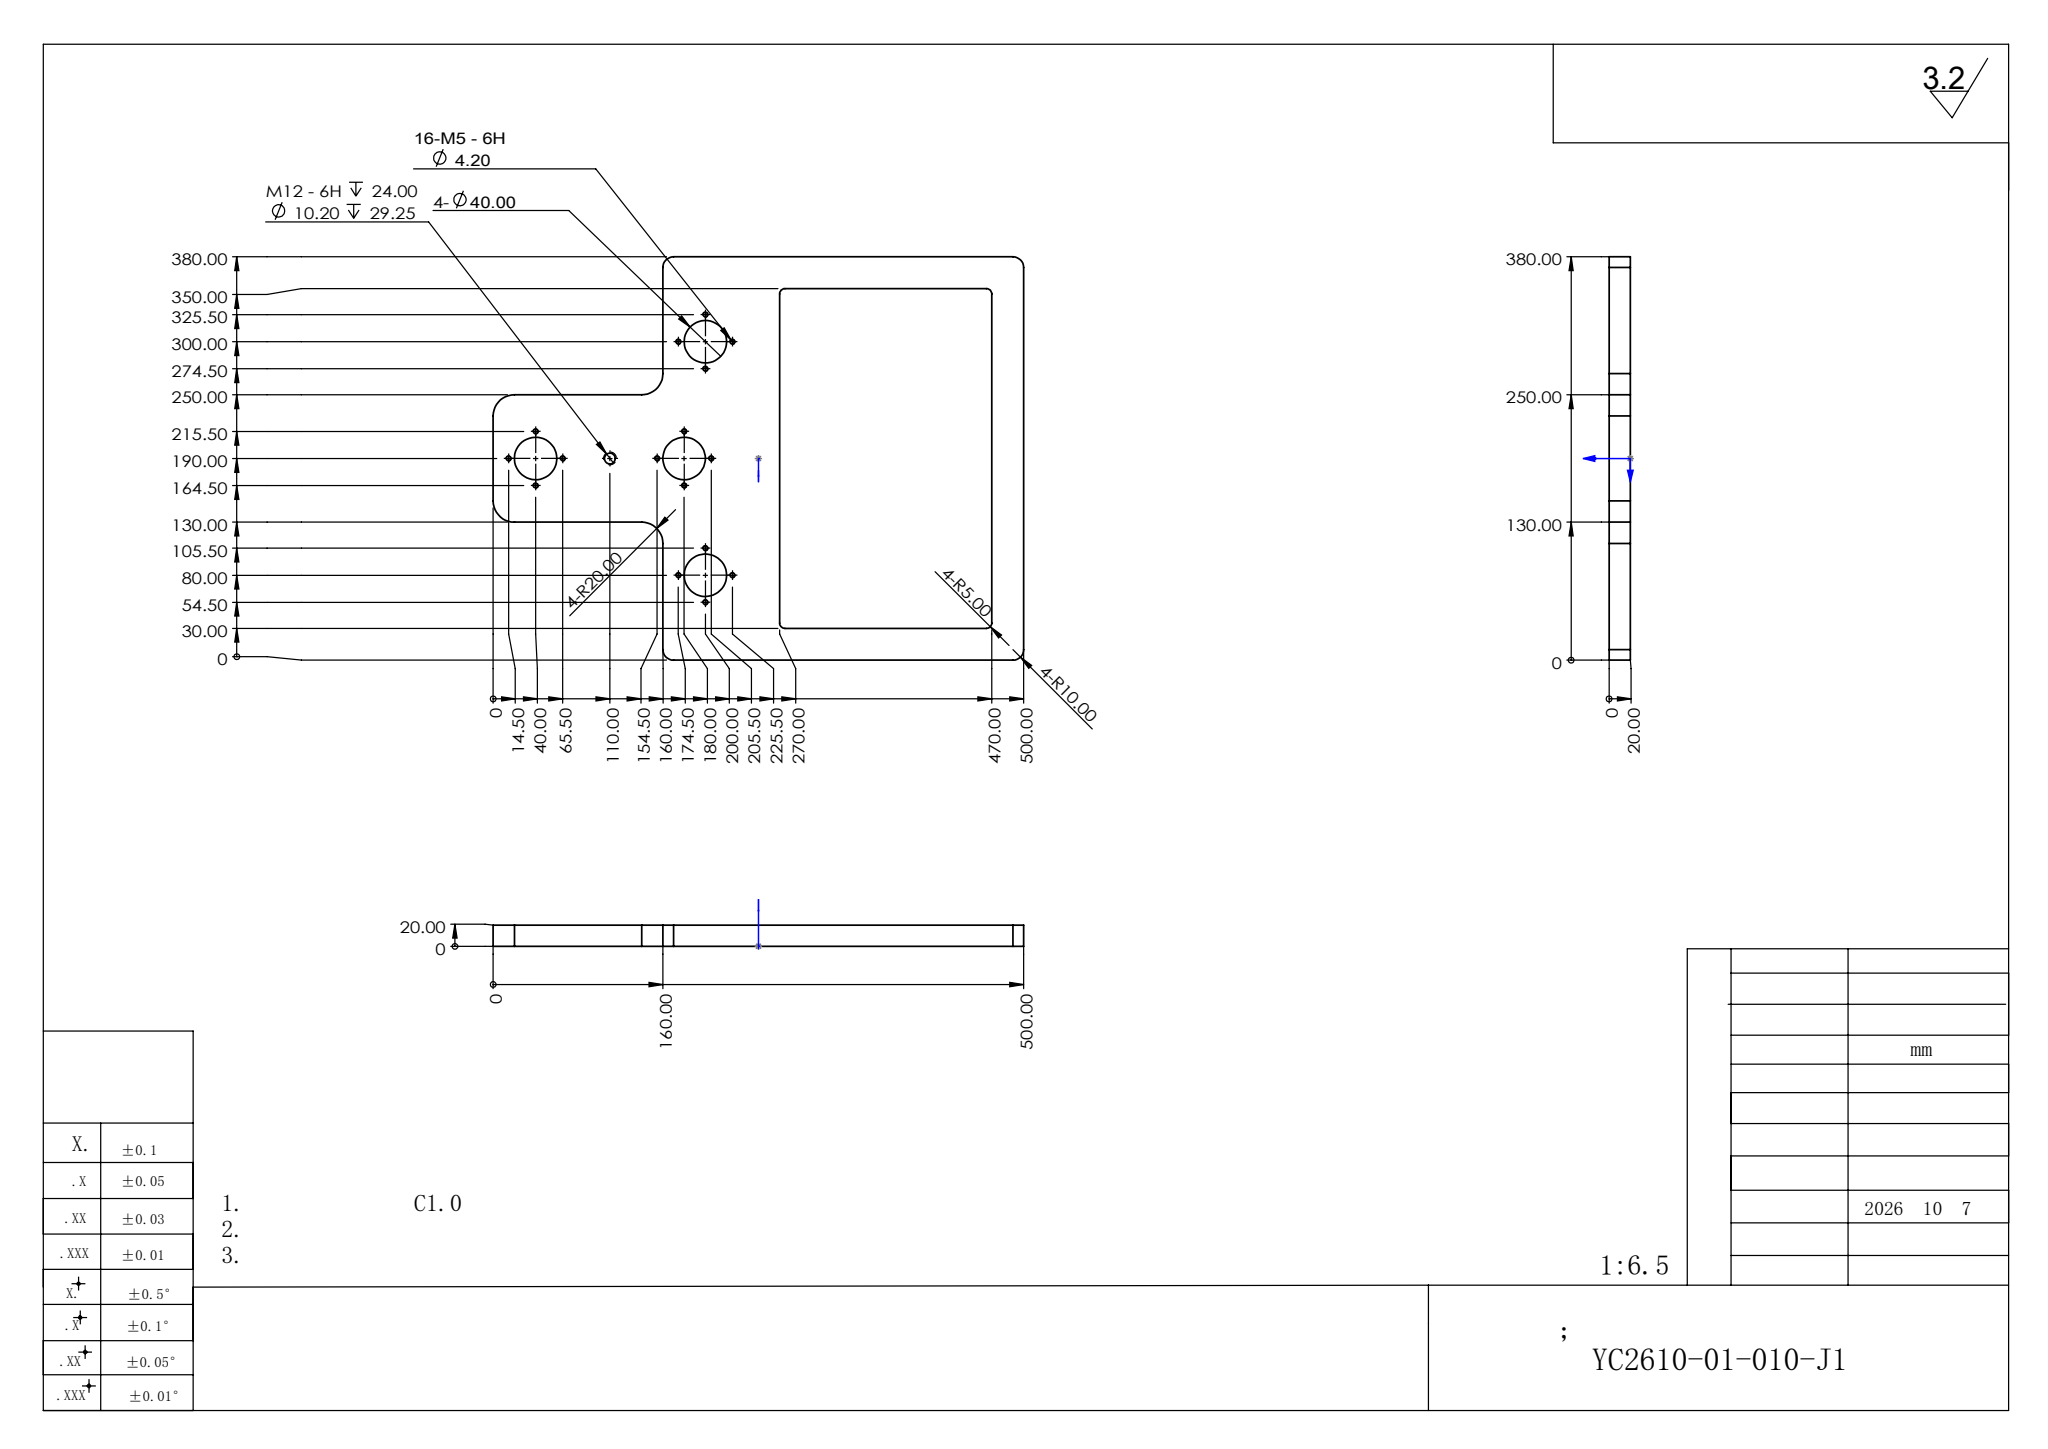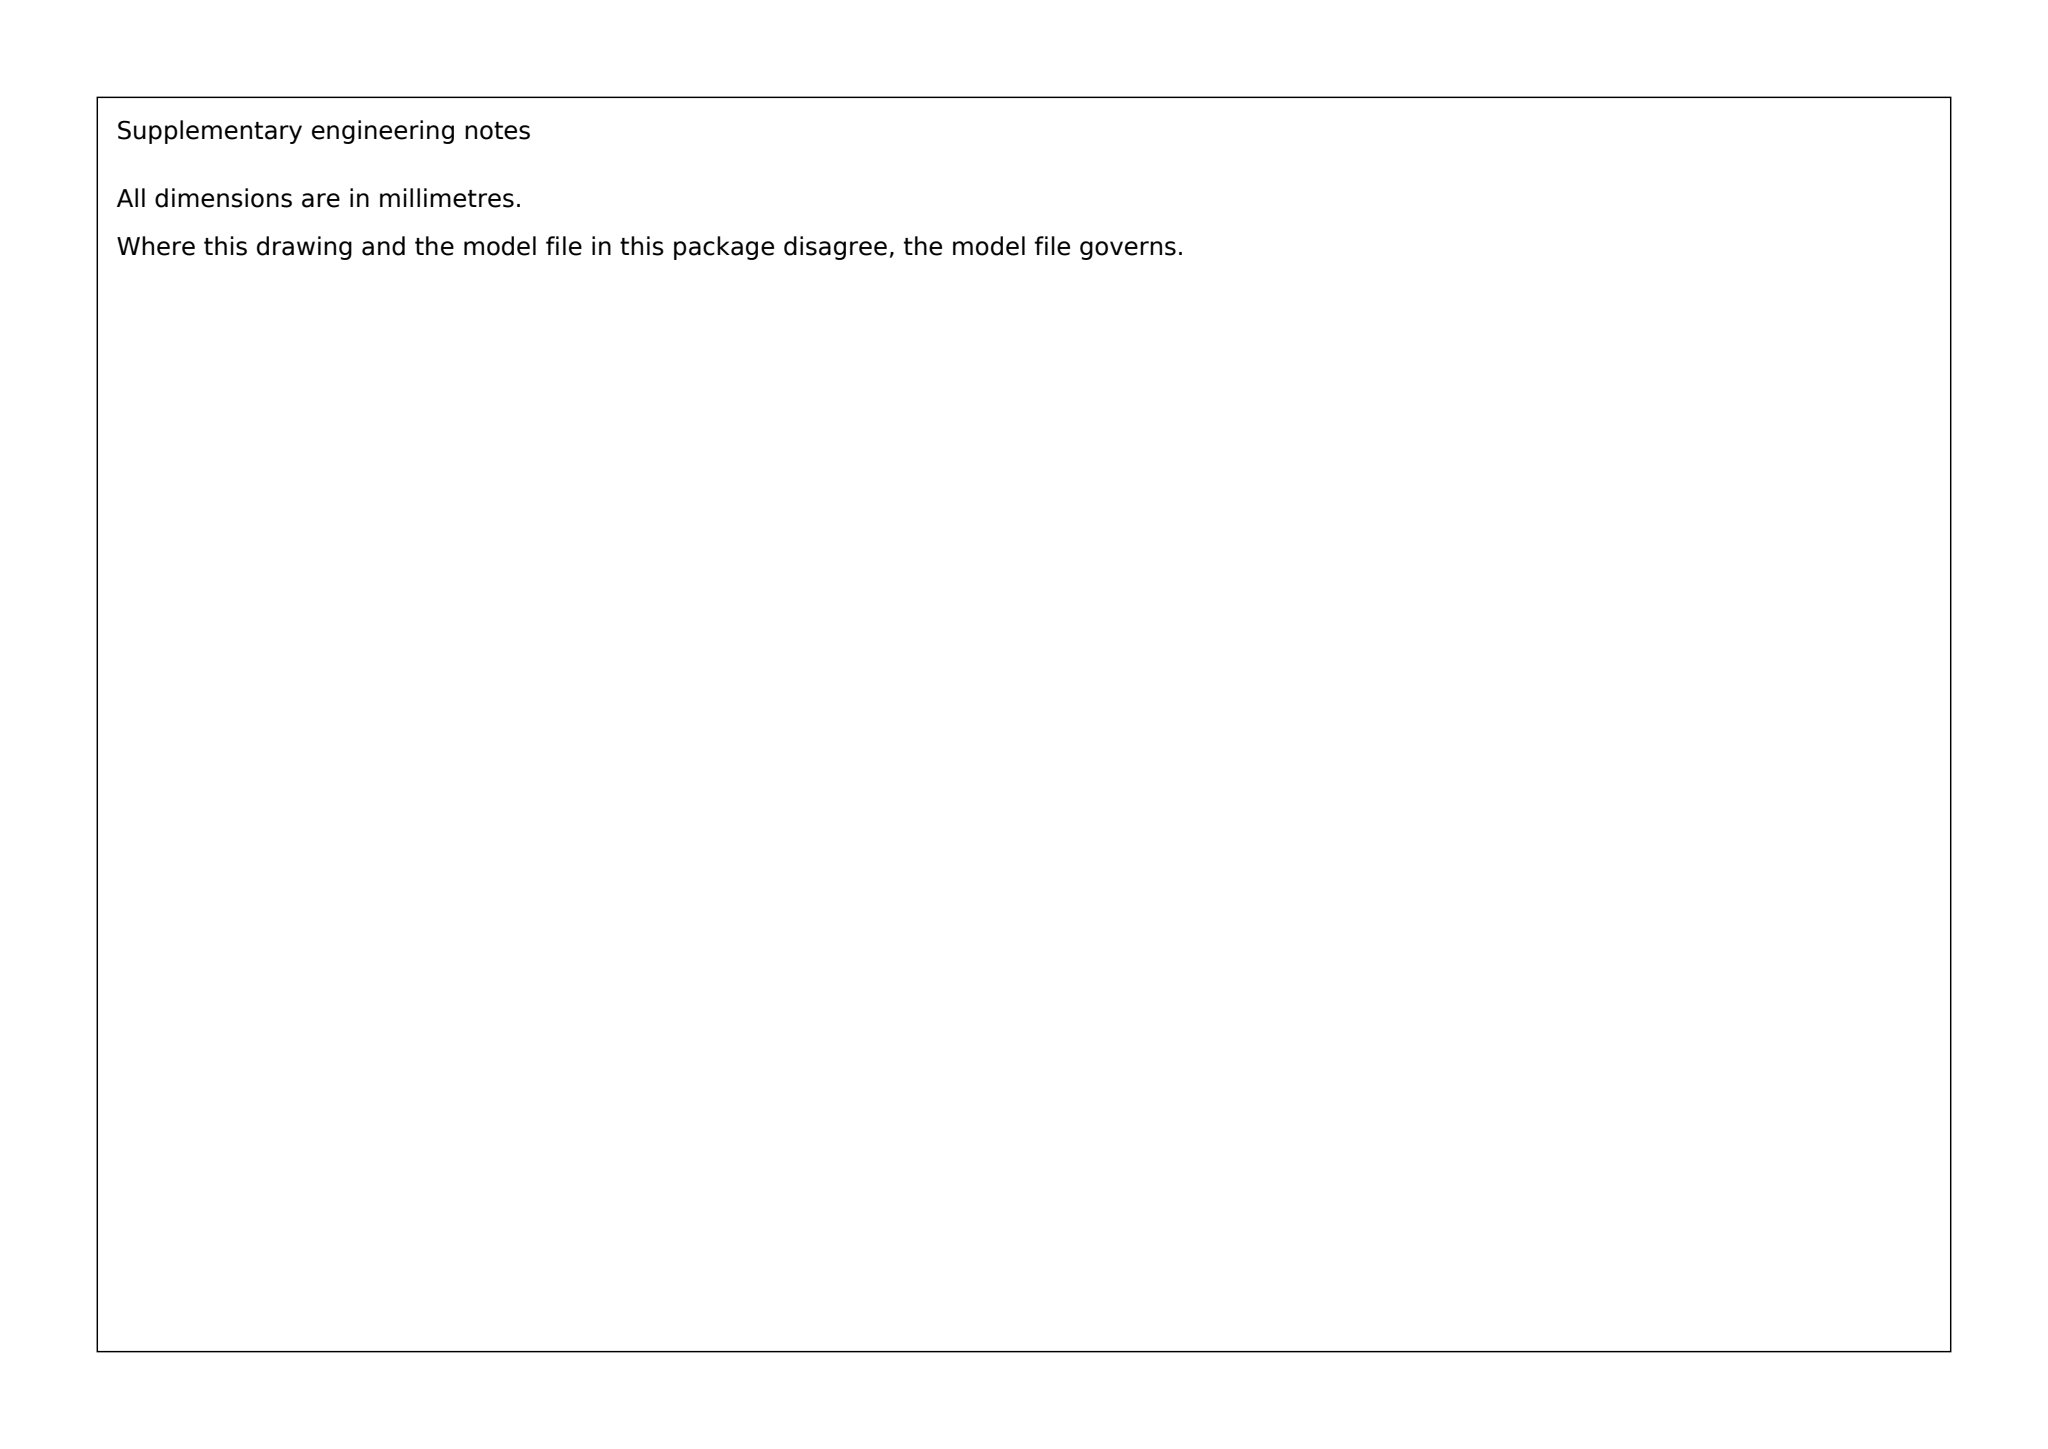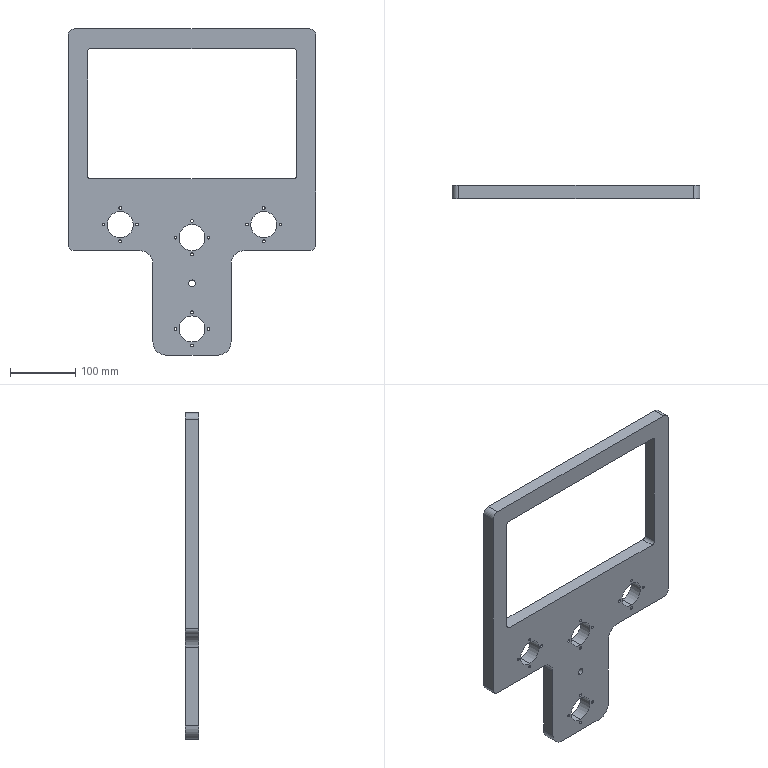Part | SolidWorks | mm | 1 solid | 68 faces | box 380 x 20 x 500 mm | volume 1580114 mm3 | cylinder 54 | plane 14 | commonest cylinder face diameters 4.2 x32 40 x12 20 x4 10 x4 10.2 x2
build123d program:
from build123d import *

# Parameters (mm, degrees)
SKETCH1_W              = 380
SKETCH1_H              = 500
BOSS_EXTRUDE1_DEPTH    = 20
SKETCH2_W              = 130
SKETCH2_H              = 160
CUT_EXTRUDE1_DEPTH     = 315.643
SKETCH3_W              = 320
SKETCH3_H              = 200
CUT_EXTRUDE2_DEPTH     = 315.643
SKETCH4_R              = 20
CUT_EXTRUDE3_DEPTH     = 315.643
M5_TAPPED_HOLE1_D      = 4.2
FILLET1_R              = 10
FILLET2_R              = 20
FILLET3_R              = 5
M12_TAPPED_HOLE1_D     = 10.2
M12_TAPPED_HOLE1_DEPTH = 29.25
M12_TAPPED_HOLE1_TIP   = 3.064


with BuildPart() as part:
    # Sketch1 → Boss-Extrude1 (new body)
    with BuildSketch(Plane(origin=(0, 0, 0), x_dir=(1, 0, 0), z_dir=(0, 1, 0))):
        Rectangle(SKETCH1_W, SKETCH1_H)
    extrude(amount=BOSS_EXTRUDE1_DEPTH)

    # Sketch2 → Cut-Extrude1 (cut, through all)
    with BuildSketch(Plane(origin=(0, 20, 0), x_dir=(1, 0, 0), z_dir=(0, 1, 0))):
        with Locations((-125, 170)):
            Rectangle(SKETCH2_W, SKETCH2_H)
        with Locations((125, 170)):
            Rectangle(SKETCH2_W, SKETCH2_H)
    extrude(amount=-CUT_EXTRUDE1_DEPTH, mode=Mode.SUBTRACT)

    # Sketch3 → Cut-Extrude2 (cut, through all)
    with BuildSketch(Plane(origin=(0, 20, 0), x_dir=(1, 0, 0), z_dir=(0, 1, 0))):
        with Locations((0, -120)):
            Rectangle(SKETCH3_W, SKETCH3_H)
    extrude(amount=-CUT_EXTRUDE2_DEPTH, mode=Mode.SUBTRACT)

    # Sketch4 → Cut-Extrude3 (cut, through all)
    with BuildSketch(Plane(origin=(0, 20, 0), x_dir=(1, 0, 0), z_dir=(0, 1, 0))):
        with Locations(Location((0, 210, 0), (0, 0, 270))):
            Circle(SKETCH4_R)
        with Locations(Location((-110, 50, 0), (0, 0, 270))):
            Circle(SKETCH4_R)
        with Locations(Location((110, 50, 0), (0, 0, 270))):
            Circle(SKETCH4_R)
        with Locations(Location((0, 70, 0), (0, 0, 270))):
            Circle(SKETCH4_R)
    extrude(amount=-CUT_EXTRUDE3_DEPTH, mode=Mode.SUBTRACT)

    # M5 Tapped Hole1 (through all)
    with Locations(Plane(origin=(0, 20, 0), x_dir=(1, 0, 0), z_dir=(0, 1, 0))):
        with Locations((0, 235.5), (0, 184.5), (25.5, 210), (-25.5, 210), (-110, 75.5), (-110, 24.5), (-84.5, 50), (-135.5, 50), (135.5, 50), (84.5, 50), (110, 75.5), (110, 24.5), (0, 95.5), (25.5, 70), (0, 44.5), (-25.5, 70)):
            Hole(M5_TAPPED_HOLE1_D / 2)

    # Fillet1
    fillet1_edges = [part.edges().sort_by_distance(p)[0] for p in [
        (-190, 10, -90),
        (190, 10, -90),
        (190, 10, 250),
        (-190, 10, 250),
    ]]
    fillet(fillet1_edges, radius=FILLET1_R)

    # Fillet2
    fillet2_edges = [part.edges().sort_by_distance(p)[0] for p in [
        (-60, 10, -250),
        (-60, 10, -90),
        (60, 10, -90),
        (60, 10, -250),
    ]]
    fillet(fillet2_edges, radius=FILLET2_R)

    # Fillet3
    fillet3_edges = [part.edges().sort_by_distance(p)[0] for p in [
        (160, 10, 20),
        (160, 10, 220),
        (-160, 10, 220),
        (-160, 10, 20),
    ]]
    fillet(fillet3_edges, radius=FILLET3_R)

    # M12 Tapped Hole1
    with Locations(Plane(origin=(0, 20, 0), x_dir=(1, 0, 0), z_dir=(0, 1, 0))):
        with Locations((0, 140)):
            Hole(M12_TAPPED_HOLE1_D / 2, depth=M12_TAPPED_HOLE1_DEPTH)
            with Locations((0, 0, -(M12_TAPPED_HOLE1_DEPTH + M12_TAPPED_HOLE1_TIP / 2))):  # 118° drill point
                Cone(0, M12_TAPPED_HOLE1_D / 2, M12_TAPPED_HOLE1_TIP, mode=Mode.SUBTRACT)


solid = part.part